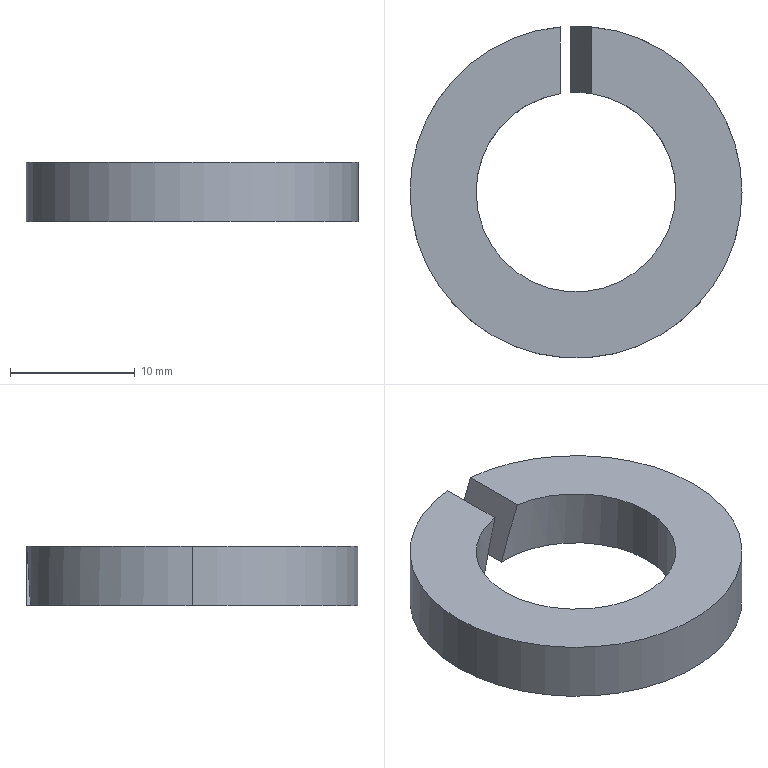Component | SolidWorks | single coil spring lock washers heavy gb-2 | 1 solid | 10 faces | box 26.6 x 26.6 x 4.8 mm | volume 1637 mm3 | cylinder 6 | plane 4 | commonest cylinder face diameters 16 x3 26.6 x3
build123d program:
from build123d import *

# Parameters (mm, degrees)
SKETCH1_R          = 13.3
SKETCH1_R_2        = 8
BASE_EXTRUDE_DEPTH = 4.8
CUT_EXTRUDE1_DEPTH = 22.197


with BuildPart() as part:
    # Sketch1 → Base-Extrude (new body)
    with BuildSketch(Plane.XY):
        Circle(SKETCH1_R)
        Circle(SKETCH1_R_2, mode=Mode.SUBTRACT)
    extrude(amount=-BASE_EXTRUDE_DEPTH)

    # Sketch2 → Cut-Extrude1 (cut, through all)
    with BuildSketch(Plane(origin=(-3.022, 0, -2.345), x_dir=(0, 0, -1), z_dir=(0, 1, 0))):
        Polygon((-2.345, -1.745), (2.455, 0.00244), (2.455, -2.552), (-2.345, -4.299), align=None)
    extrude(amount=CUT_EXTRUDE1_DEPTH, mode=Mode.SUBTRACT)


solid = part.part

# Placed as in the assembly
solid = solid.moved(Location((0, 14, -25), (0, 0, 0)))
STEP:
#1=CARTESIAN_POINT('',(-0.315,0.5512,-1.173));
#2=VERTEX_POINT('',#1);
#3=CARTESIAN_POINT('',(0.315,0.5512,-1.173));
#4=VERTEX_POINT('',#3);
#5=CARTESIAN_POINT('',(0.,0.5512,-1.173));
#6=DIRECTION('',(0.,0.,1.));
#7=DIRECTION('',(1.,0.,0.));
#8=AXIS2_PLACEMENT_3D('',#5,#6,#7);
#9=CIRCLE('',#8,0.315);
#10=EDGE_CURVE('',#2,#4,#9,.T.);
#11=ORIENTED_EDGE('',*,*,#10,.F.);
#12=CARTESIAN_POINT('',(-0.315,0.5512,-0.9843));
#13=VERTEX_POINT('',#12);
#14=CARTESIAN_POINT('',(-0.315,0.5512,-1.173));
#15=DIRECTION('',(0.,0.,1.));
#16=VECTOR('',#15,39.37);
#17=LINE('',#14,#16);
#18=EDGE_CURVE('',#2,#13,#17,.T.);
#19=ORIENTED_EDGE('',*,*,#18,.T.);
#20=CARTESIAN_POINT('',(0.315,0.5512,-0.9843));
#21=VERTEX_POINT('',#20);
#22=CARTESIAN_POINT('',(0.,0.5512,-0.9843));
#23=DIRECTION('',(0.,0.,1.));
#24=DIRECTION('',(1.,0.,0.));
#25=AXIS2_PLACEMENT_3D('',#22,#23,#24);
#26=CIRCLE('',#25,0.315);
#27=EDGE_CURVE('',#13,#21,#26,.T.);
#28=ORIENTED_EDGE('',*,*,#27,.T.);
#29=CARTESIAN_POINT('',(0.315,0.5512,-1.173));
#30=DIRECTION('',(0.,0.,1.));
#31=VECTOR('',#30,39.37);
#32=LINE('',#29,#31);
#33=EDGE_CURVE('',#4,#21,#32,.T.);
#34=ORIENTED_EDGE('',*,*,#33,.F.);
#35=EDGE_LOOP('',(#11,#19,#28,#34));
#36=FACE_OUTER_BOUND('',#35,.T.);
#37=CARTESIAN_POINT('',(0.,0.5512,-1.173));
#38=DIRECTION('',(0.,0.,1.));
#39=DIRECTION('',(1.,0.,0.));
#40=AXIS2_PLACEMENT_3D('',#37,#38,#39);
#41=CYLINDRICAL_SURFACE('',#40,0.315);
#42=ADVANCED_FACE('',(#36),#41,.F.);
#43=CARTESIAN_POINT('',(-0.01851,0.8656,-1.173));
#44=VERTEX_POINT('',#43);
#45=CARTESIAN_POINT('',(0.,0.5512,-1.173));
#46=DIRECTION('',(0.,0.,1.));
#47=DIRECTION('',(1.,0.,0.));
#48=AXIS2_PLACEMENT_3D('',#45,#46,#47);
#49=CIRCLE('',#48,0.315);
#50=EDGE_CURVE('',#4,#44,#49,.T.);
#51=ORIENTED_EDGE('',*,*,#50,.F.);
#52=ORIENTED_EDGE('',*,*,#33,.T.);
#53=CARTESIAN_POINT('',(0.05028,0.8621,-0.9843));
#54=VERTEX_POINT('',#53);
#55=CARTESIAN_POINT('',(0.,0.5512,-0.9843));
#56=DIRECTION('',(0.,0.,1.));
#57=DIRECTION('',(1.,0.,0.));
#58=AXIS2_PLACEMENT_3D('',#55,#56,#57);
#59=CIRCLE('',#58,0.315);
#60=EDGE_CURVE('',#21,#54,#59,.T.);
#61=ORIENTED_EDGE('',*,*,#60,.T.);
#62=CARTESIAN_POINT('',(-0.01851,0.8656,-1.173));
#63=CARTESIAN_POINT('',(0.004503,0.867,-1.11));
#64=CARTESIAN_POINT('',(0.02752,0.8658,-1.047));
#65=CARTESIAN_POINT('',(0.05028,0.8621,-0.9843));
#66=(BOUNDED_CURVE()B_SPLINE_CURVE(3,(#62,#63,#64,#65),.UNSPECIFIED.,.F.,.T.)B_SPLINE_CURVE_WITH_KNOTS((4,4),(4.654,4.873),.UNSPECIFIED.)CURVE()GEOMETRIC_REPRESENTATION_ITEM()RATIONAL_B_SPLINE_CURVE((1.,0.996,0.996,1.))REPRESENTATION_ITEM(''));
#67=EDGE_CURVE('',#44,#54,#66,.T.);
#68=ORIENTED_EDGE('',*,*,#67,.F.);
#69=EDGE_LOOP('',(#51,#52,#61,#68));
#70=FACE_OUTER_BOUND('',#69,.T.);
#71=CARTESIAN_POINT('',(0.,0.5512,-1.173));
#72=DIRECTION('',(0.,0.,1.));
#73=DIRECTION('',(1.,0.,0.));
#74=AXIS2_PLACEMENT_3D('',#71,#72,#73);
#75=CYLINDRICAL_SURFACE('',#74,0.315);
#76=ADVANCED_FACE('',(#70),#75,.F.);
#77=CARTESIAN_POINT('',(-0.1191,1.061,-1.173));
#78=VERTEX_POINT('',#77);
#79=CARTESIAN_POINT('',(-0.5236,0.5512,-1.173));
#80=VERTEX_POINT('',#79);
#81=CARTESIAN_POINT('',(0.,0.5512,-1.173));
#82=DIRECTION('',(0.,0.,1.));
#83=DIRECTION('',(1.,0.,0.));
#84=AXIS2_PLACEMENT_3D('',#81,#82,#83);
#85=CIRCLE('',#84,0.5236);
#86=EDGE_CURVE('',#78,#80,#85,.T.);
#87=ORIENTED_EDGE('',*,*,#86,.T.);
#88=CARTESIAN_POINT('',(-0.5236,0.5512,-0.9843));
#89=VERTEX_POINT('',#88);
#90=CARTESIAN_POINT('',(-0.5236,0.5512,-1.173));
#91=DIRECTION('',(0.,0.,1.));
#92=VECTOR('',#91,39.37);
#93=LINE('',#90,#92);
#94=EDGE_CURVE('',#80,#89,#93,.T.);
#95=ORIENTED_EDGE('',*,*,#94,.T.);
#96=CARTESIAN_POINT('',(-0.05028,1.072,-0.9843));
#97=VERTEX_POINT('',#96);
#98=CARTESIAN_POINT('',(0.,0.5512,-0.9843));
#99=DIRECTION('',(0.,0.,1.));
#100=DIRECTION('',(1.,0.,0.));
#101=AXIS2_PLACEMENT_3D('',#98,#99,#100);
#102=CIRCLE('',#101,0.5236);
#103=EDGE_CURVE('',#97,#89,#102,.T.);
#104=ORIENTED_EDGE('',*,*,#103,.F.);
#105=CARTESIAN_POINT('',(-0.05028,1.072,-0.9843));
#106=CARTESIAN_POINT('',(-0.07344,1.07,-1.048));
#107=CARTESIAN_POINT('',(-0.0964,1.066,-1.111));
#108=CARTESIAN_POINT('',(-0.1191,1.061,-1.173));
#109=(BOUNDED_CURVE()B_SPLINE_CURVE(3,(#105,#106,#107,#108),.UNSPECIFIED.,.F.,.T.)B_SPLINE_CURVE_WITH_KNOTS((4,4),(1.667,1.8),.UNSPECIFIED.)CURVE()GEOMETRIC_REPRESENTATION_ITEM()RATIONAL_B_SPLINE_CURVE((1.,0.9985,0.9985,1.))REPRESENTATION_ITEM(''));
#110=EDGE_CURVE('',#97,#78,#109,.T.);
#111=ORIENTED_EDGE('',*,*,#110,.T.);
#112=EDGE_LOOP('',(#87,#95,#104,#111));
#113=FACE_OUTER_BOUND('',#112,.T.);
#114=CARTESIAN_POINT('',(0.,0.5512,-1.173));
#115=DIRECTION('',(0.,0.,1.));
#116=DIRECTION('',(1.,0.,0.));
#117=AXIS2_PLACEMENT_3D('',#114,#115,#116);
#118=CYLINDRICAL_SURFACE('',#117,0.5236);
#119=ADVANCED_FACE('',(#113),#118,.T.);
#120=ORIENTED_EDGE('',*,*,#94,.F.);
#121=CARTESIAN_POINT('',(0.5236,0.5512,-1.173));
#122=VERTEX_POINT('',#121);
#123=CARTESIAN_POINT('',(0.,0.5512,-1.173));
#124=DIRECTION('',(0.,0.,1.));
#125=DIRECTION('',(1.,0.,0.));
#126=AXIS2_PLACEMENT_3D('',#123,#124,#125);
#127=CIRCLE('',#126,0.5236);
#128=EDGE_CURVE('',#80,#122,#127,.T.);
#129=ORIENTED_EDGE('',*,*,#128,.T.);
#130=CARTESIAN_POINT('',(0.5236,0.5512,-0.9843));
#131=VERTEX_POINT('',#130);
#132=CARTESIAN_POINT('',(0.5236,0.5512,-1.173));
#133=DIRECTION('',(0.,0.,1.));
#134=VECTOR('',#133,39.37);
#135=LINE('',#132,#134);
#136=EDGE_CURVE('',#122,#131,#135,.T.);
#137=ORIENTED_EDGE('',*,*,#136,.T.);
#138=CARTESIAN_POINT('',(0.,0.5512,-0.9843));
#139=DIRECTION('',(0.,0.,1.));
#140=DIRECTION('',(1.,0.,0.));
#141=AXIS2_PLACEMENT_3D('',#138,#139,#140);
#142=CIRCLE('',#141,0.5236);
#143=EDGE_CURVE('',#89,#131,#142,.T.);
#144=ORIENTED_EDGE('',*,*,#143,.F.);
#145=EDGE_LOOP('',(#120,#129,#137,#144));
#146=FACE_OUTER_BOUND('',#145,.T.);
#147=CARTESIAN_POINT('',(0.,0.5512,-1.173));
#148=DIRECTION('',(0.,0.,1.));
#149=DIRECTION('',(1.,0.,0.));
#150=AXIS2_PLACEMENT_3D('',#147,#148,#149);
#151=CYLINDRICAL_SURFACE('',#150,0.5236);
#152=ADVANCED_FACE('',(#146),#151,.T.);
#153=ORIENTED_EDGE('',*,*,#136,.F.);
#154=CARTESIAN_POINT('',(-0.01851,1.074,-1.173));
#155=VERTEX_POINT('',#154);
#156=CARTESIAN_POINT('',(0.,0.5512,-1.173));
#157=DIRECTION('',(0.,0.,1.));
#158=DIRECTION('',(1.,0.,0.));
#159=AXIS2_PLACEMENT_3D('',#156,#157,#158);
#160=CIRCLE('',#159,0.5236);
#161=EDGE_CURVE('',#122,#155,#160,.T.);
#162=ORIENTED_EDGE('',*,*,#161,.T.);
#163=CARTESIAN_POINT('',(0.05028,1.072,-0.9843));
#164=VERTEX_POINT('',#163);
#165=CARTESIAN_POINT('',(-0.01851,1.074,-1.173));
#166=CARTESIAN_POINT('',(0.004451,1.075,-1.11));
#167=CARTESIAN_POINT('',(0.02741,1.075,-1.047));
#168=CARTESIAN_POINT('',(0.05028,1.072,-0.9843));
#169=(BOUNDED_CURVE()B_SPLINE_CURVE(3,(#165,#166,#167,#168),.UNSPECIFIED.,.F.,.F.)B_SPLINE_CURVE_WITH_KNOTS((4,4),(4.677,4.809),.UNSPECIFIED.)CURVE()GEOMETRIC_REPRESENTATION_ITEM()RATIONAL_B_SPLINE_CURVE((1.,0.9986,0.9986,1.))REPRESENTATION_ITEM(''));
#170=EDGE_CURVE('',#155,#164,#169,.T.);
#171=ORIENTED_EDGE('',*,*,#170,.T.);
#172=CARTESIAN_POINT('',(0.,0.5512,-0.9843));
#173=DIRECTION('',(0.,0.,1.));
#174=DIRECTION('',(1.,0.,0.));
#175=AXIS2_PLACEMENT_3D('',#172,#173,#174);
#176=CIRCLE('',#175,0.5236);
#177=EDGE_CURVE('',#131,#164,#176,.T.);
#178=ORIENTED_EDGE('',*,*,#177,.F.);
#179=EDGE_LOOP('',(#153,#162,#171,#178));
#180=FACE_OUTER_BOUND('',#179,.T.);
#181=CARTESIAN_POINT('',(0.,0.5512,-1.173));
#182=DIRECTION('',(0.,0.,1.));
#183=DIRECTION('',(1.,0.,0.));
#184=AXIS2_PLACEMENT_3D('',#181,#182,#183);
#185=CYLINDRICAL_SURFACE('',#184,0.5236);
#186=ADVANCED_FACE('',(#180),#185,.T.);
#187=CARTESIAN_POINT('',(-0.01851,1.075,-1.173));
#188=DIRECTION('',(0.,-1.,0.));
#189=VECTOR('',#188,39.37);
#190=LINE('',#187,#189);
#191=EDGE_CURVE('',#155,#44,#190,.T.);
#192=ORIENTED_EDGE('',*,*,#191,.F.);
#193=ORIENTED_EDGE('',*,*,#161,.F.);
#194=ORIENTED_EDGE('',*,*,#128,.F.);
#195=ORIENTED_EDGE('',*,*,#86,.F.);
#196=CARTESIAN_POINT('',(-0.1191,0.8428,-1.173));
#197=VERTEX_POINT('',#196);
#198=CARTESIAN_POINT('',(-0.1191,1.075,-1.173));
#199=DIRECTION('',(0.,-1.,0.));
#200=VECTOR('',#199,39.37);
#201=LINE('',#198,#200);
#202=EDGE_CURVE('',#78,#197,#201,.T.);
#203=ORIENTED_EDGE('',*,*,#202,.T.);
#204=CARTESIAN_POINT('',(0.,0.5512,-1.173));
#205=DIRECTION('',(0.,0.,1.));
#206=DIRECTION('',(1.,0.,0.));
#207=AXIS2_PLACEMENT_3D('',#204,#205,#206);
#208=CIRCLE('',#207,0.315);
#209=EDGE_CURVE('',#197,#2,#208,.T.);
#210=ORIENTED_EDGE('',*,*,#209,.T.);
#211=ORIENTED_EDGE('',*,*,#10,.T.);
#212=ORIENTED_EDGE('',*,*,#50,.T.);
#213=EDGE_LOOP('',(#192,#193,#194,#195,#203,#210,#211,#212));
#214=FACE_OUTER_BOUND('',#213,.T.);
#215=CARTESIAN_POINT('',(0.,0.5512,-1.173));
#216=DIRECTION('',(0.,0.,1.));
#217=DIRECTION('',(1.,0.,0.));
#218=AXIS2_PLACEMENT_3D('',#215,#216,#217);
#219=PLANE('',#218);
#220=ADVANCED_FACE('',(#214),#219,.F.);
#221=ORIENTED_EDGE('',*,*,#103,.T.);
#222=ORIENTED_EDGE('',*,*,#143,.T.);
#223=ORIENTED_EDGE('',*,*,#177,.T.);
#224=CARTESIAN_POINT('',(0.05028,1.075,-0.9843));
#225=DIRECTION('',(0.,-1.,0.));
#226=VECTOR('',#225,39.37);
#227=LINE('',#224,#226);
#228=EDGE_CURVE('',#164,#54,#227,.T.);
#229=ORIENTED_EDGE('',*,*,#228,.T.);
#230=ORIENTED_EDGE('',*,*,#60,.F.);
#231=ORIENTED_EDGE('',*,*,#27,.F.);
#232=CARTESIAN_POINT('',(-0.05028,0.8621,-0.9843));
#233=VERTEX_POINT('',#232);
#234=CARTESIAN_POINT('',(0.,0.5512,-0.9843));
#235=DIRECTION('',(0.,0.,1.));
#236=DIRECTION('',(1.,0.,0.));
#237=AXIS2_PLACEMENT_3D('',#234,#235,#236);
#238=CIRCLE('',#237,0.315);
#239=EDGE_CURVE('',#233,#13,#238,.T.);
#240=ORIENTED_EDGE('',*,*,#239,.F.);
#241=CARTESIAN_POINT('',(-0.05028,1.075,-0.9843));
#242=DIRECTION('',(0.,-1.,0.));
#243=VECTOR('',#242,39.37);
#244=LINE('',#241,#243);
#245=EDGE_CURVE('',#97,#233,#244,.T.);
#246=ORIENTED_EDGE('',*,*,#245,.F.);
#247=EDGE_LOOP('',(#221,#222,#223,#229,#230,#231,#240,#246));
#248=FACE_OUTER_BOUND('',#247,.T.);
#249=CARTESIAN_POINT('',(0.,0.5512,-0.9843));
#250=DIRECTION('',(0.,0.,1.));
#251=DIRECTION('',(1.,0.,0.));
#252=AXIS2_PLACEMENT_3D('',#249,#250,#251);
#253=PLANE('',#252);
#254=ADVANCED_FACE('',(#248),#253,.T.);
#255=ORIENTED_EDGE('',*,*,#18,.F.);
#256=ORIENTED_EDGE('',*,*,#209,.F.);
#257=CARTESIAN_POINT('',(-0.05028,0.8621,-0.9843));
#258=CARTESIAN_POINT('',(-0.07389,0.8583,-1.049));
#259=CARTESIAN_POINT('',(-0.09691,0.8518,-1.112));
#260=CARTESIAN_POINT('',(-0.1191,0.8428,-1.173));
#261=(BOUNDED_CURVE()B_SPLINE_CURVE(3,(#257,#258,#259,#260),.UNSPECIFIED.,.F.,.F.)B_SPLINE_CURVE_WITH_KNOTS((4,4),(1.731,1.958),.UNSPECIFIED.)CURVE()GEOMETRIC_REPRESENTATION_ITEM()RATIONAL_B_SPLINE_CURVE((1.,0.9957,0.9957,1.))REPRESENTATION_ITEM(''));
#262=EDGE_CURVE('',#233,#197,#261,.T.);
#263=ORIENTED_EDGE('',*,*,#262,.F.);
#264=ORIENTED_EDGE('',*,*,#239,.T.);
#265=EDGE_LOOP('',(#255,#256,#263,#264));
#266=FACE_OUTER_BOUND('',#265,.T.);
#267=CARTESIAN_POINT('',(0.,0.5512,-1.173));
#268=DIRECTION('',(0.,0.,1.));
#269=DIRECTION('',(1.,0.,0.));
#270=AXIS2_PLACEMENT_3D('',#267,#268,#269);
#271=CYLINDRICAL_SURFACE('',#270,0.315);
#272=ADVANCED_FACE('',(#266),#271,.F.);
#273=ORIENTED_EDGE('',*,*,#245,.T.);
#274=ORIENTED_EDGE('',*,*,#262,.T.);
#275=ORIENTED_EDGE('',*,*,#202,.F.);
#276=ORIENTED_EDGE('',*,*,#110,.F.);
#277=EDGE_LOOP('',(#273,#274,#275,#276));
#278=FACE_OUTER_BOUND('',#277,.T.);
#279=CARTESIAN_POINT('',(-0.05028,1.075,-0.9843));
#280=DIRECTION('',(0.9397,0.,-0.342));
#281=DIRECTION('',(-0.342,0.,-0.9397));
#282=AXIS2_PLACEMENT_3D('',#279,#280,#281);
#283=PLANE('',#282);
#284=ADVANCED_FACE('',(#278),#283,.T.);
#285=ORIENTED_EDGE('',*,*,#191,.T.);
#286=ORIENTED_EDGE('',*,*,#67,.T.);
#287=ORIENTED_EDGE('',*,*,#228,.F.);
#288=ORIENTED_EDGE('',*,*,#170,.F.);
#289=EDGE_LOOP('',(#285,#286,#287,#288));
#290=FACE_OUTER_BOUND('',#289,.T.);
#291=CARTESIAN_POINT('',(0.05028,1.075,-0.9843));
#292=DIRECTION('',(-0.9397,0.,0.342));
#293=DIRECTION('',(0.342,0.,0.9397));
#294=AXIS2_PLACEMENT_3D('',#291,#292,#293);
#295=PLANE('',#294);
#296=ADVANCED_FACE('',(#290),#295,.T.);
#297=CLOSED_SHELL('',(#42,#76,#119,#152,#186,#220,#254,#272,#284,#296));
#298=MANIFOLD_SOLID_BREP('',#297);
#299=CARTESIAN_POINT('',(0.,0.,0.));
#300=DIRECTION('',(0.,0.,1.));
#301=DIRECTION('',(1.,0.,0.));
#302=AXIS2_PLACEMENT_3D('',#299,#300,#301);
#303=(LENGTH_UNIT()NAMED_UNIT(*)SI_UNIT($,.METRE.));
#304=LENGTH_MEASURE_WITH_UNIT(LENGTH_MEASURE(0.0254),#303);
#305=DIMENSIONAL_EXPONENTS(1.,0.,0.,0.,0.,0.,0.);
#306=(CONVERSION_BASED_UNIT('',#304)LENGTH_UNIT()NAMED_UNIT(#305));
#307=UNCERTAINTY_MEASURE_WITH_UNIT(LENGTH_MEASURE(0.00001),#306,'','');
#308=(NAMED_UNIT(*)PLANE_ANGLE_UNIT()SI_UNIT($,.RADIAN.));
#309=(NAMED_UNIT(*)SI_UNIT($,.STERADIAN.)SOLID_ANGLE_UNIT());
#310=(GEOMETRIC_REPRESENTATION_CONTEXT(3)GLOBAL_UNCERTAINTY_ASSIGNED_CONTEXT((#307))GLOBAL_UNIT_ASSIGNED_CONTEXT((#306,#308,#309))REPRESENTATION_CONTEXT('',''));
#311=ADVANCED_BREP_SHAPE_REPRESENTATION('',(#298,#302),#310);
#312=COLOUR_RGB('',0.7922,0.8196,0.9333);
#313=FILL_AREA_STYLE_COLOUR('',#312);
#314=FILL_AREA_STYLE('',(#313));
#315=SURFACE_STYLE_FILL_AREA(#314);
#316=SURFACE_SIDE_STYLE('',(#315));
#317=SURFACE_STYLE_USAGE(.BOTH.,#316);
#318=PRESENTATION_STYLE_ASSIGNMENT((#317));
#319=STYLED_ITEM('',(#318),#298);
#320=PRESENTATION_LAYER_ASSIGNMENT('','',(#319));
#321=(LENGTH_UNIT()NAMED_UNIT(*)SI_UNIT($,.METRE.));
#322=LENGTH_MEASURE_WITH_UNIT(LENGTH_MEASURE(0.0254),#321);
#323=DIMENSIONAL_EXPONENTS(1.,0.,0.,0.,0.,0.,0.);
#324=(CONVERSION_BASED_UNIT('',#322)LENGTH_UNIT()NAMED_UNIT(#323));
#325=UNCERTAINTY_MEASURE_WITH_UNIT(LENGTH_MEASURE(0.00001),#324,'','');
#326=(NAMED_UNIT(*)PLANE_ANGLE_UNIT()SI_UNIT($,.RADIAN.));
#327=(NAMED_UNIT(*)SI_UNIT($,.STERADIAN.)SOLID_ANGLE_UNIT());
#328=(GEOMETRIC_REPRESENTATION_CONTEXT(3)GLOBAL_UNCERTAINTY_ASSIGNED_CONTEXT((#325))GLOBAL_UNIT_ASSIGNED_CONTEXT((#324,#326,#327))REPRESENTATION_CONTEXT('',''));
#329=MECHANICAL_DESIGN_GEOMETRIC_PRESENTATION_REPRESENTATION('',(#319),#328);